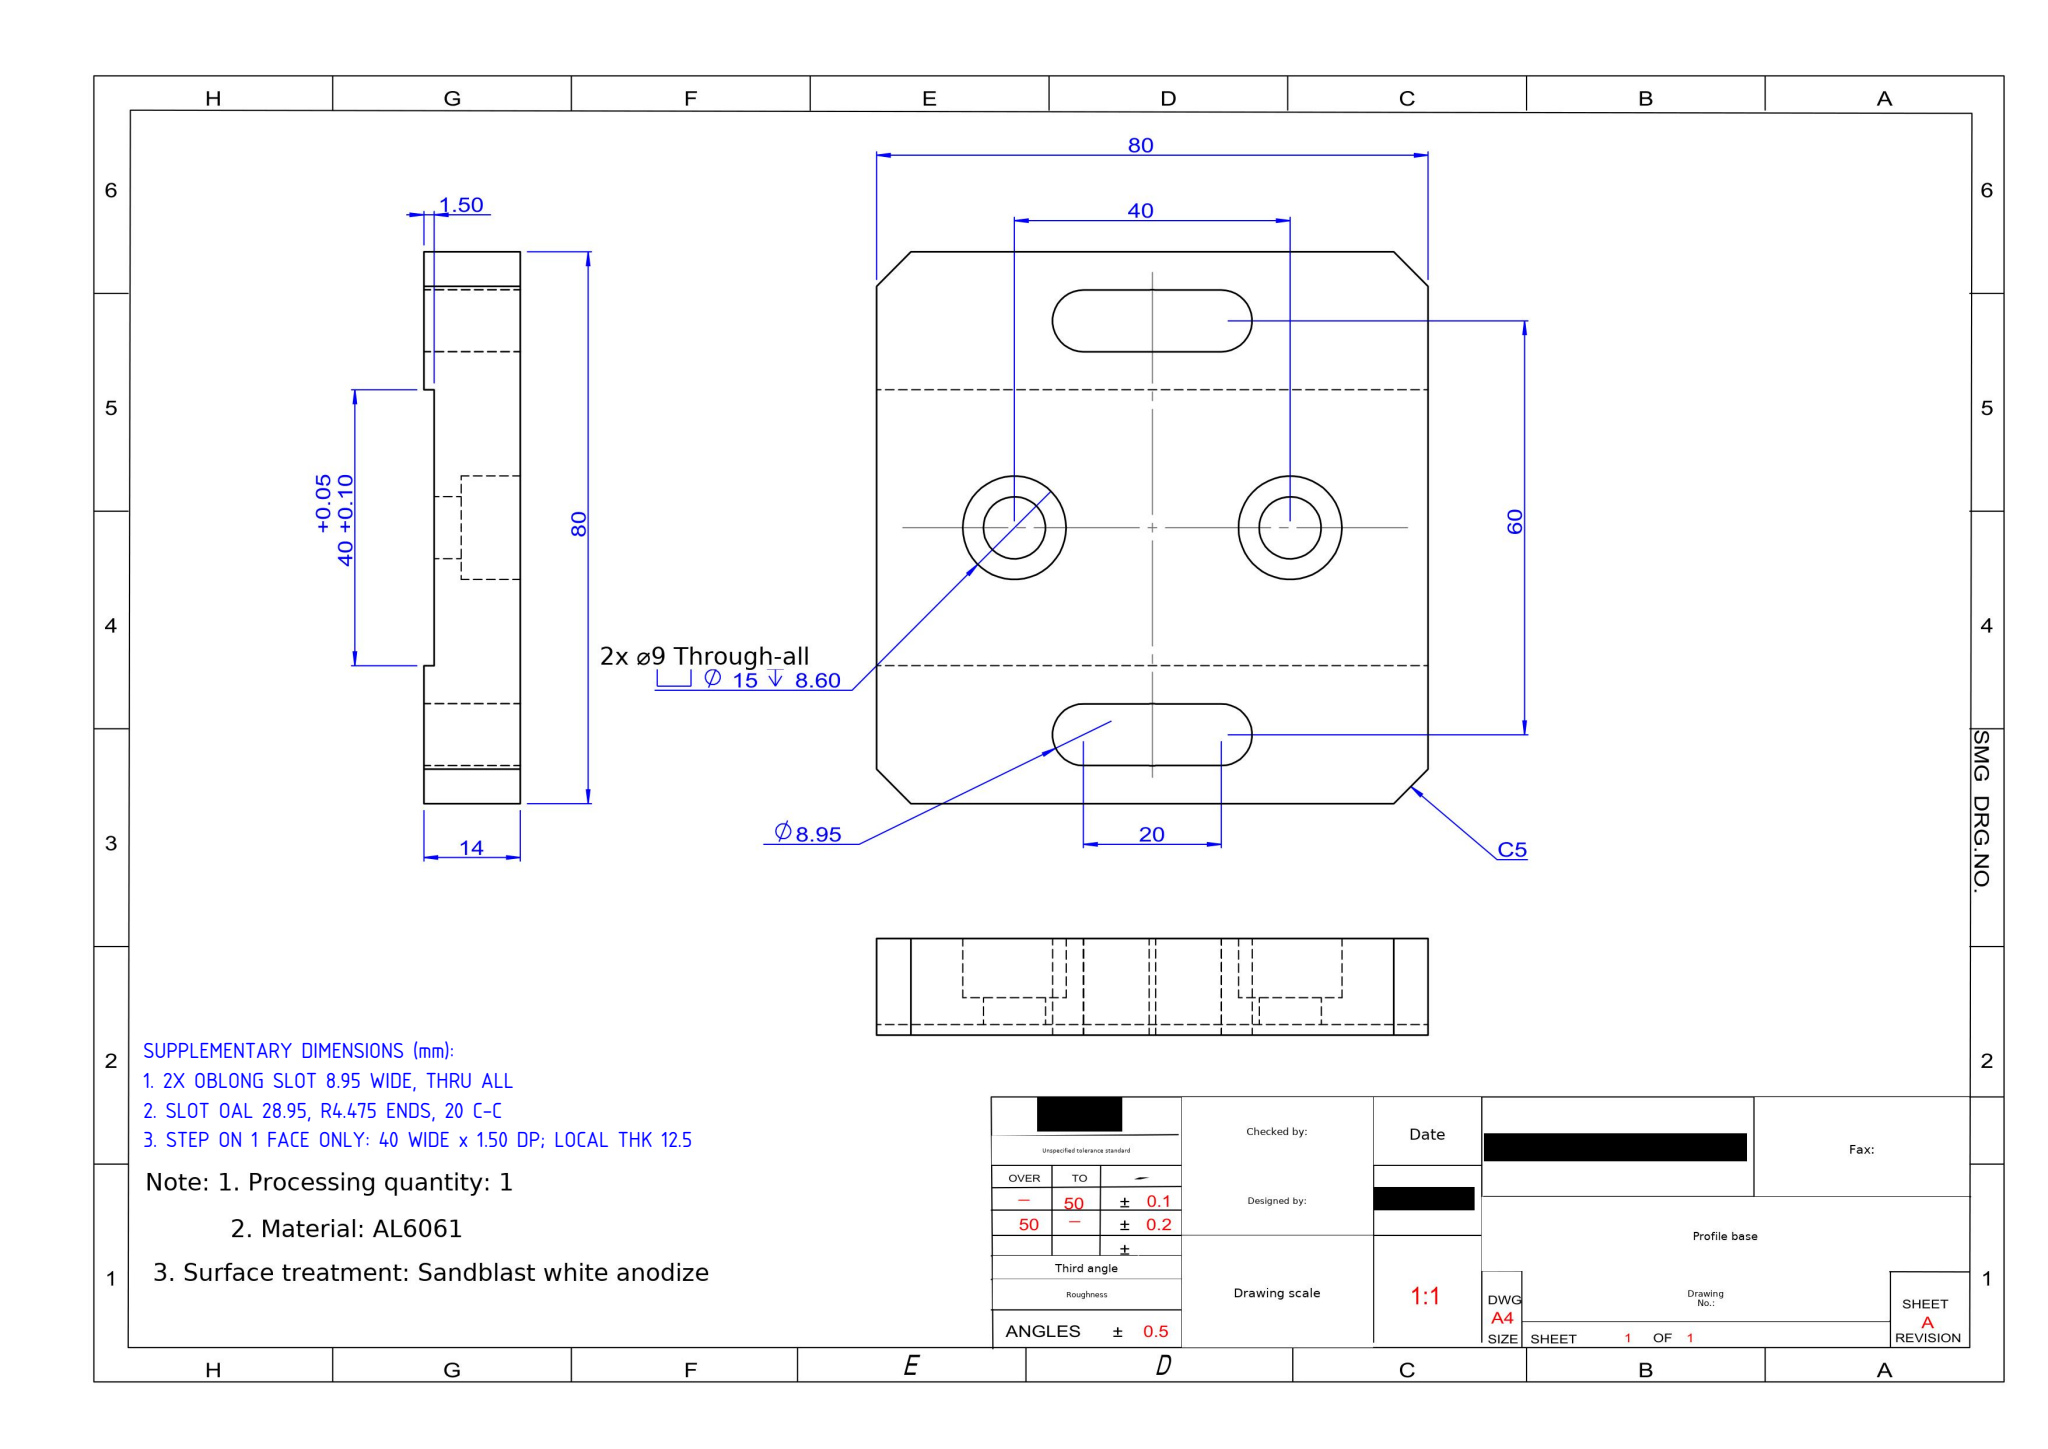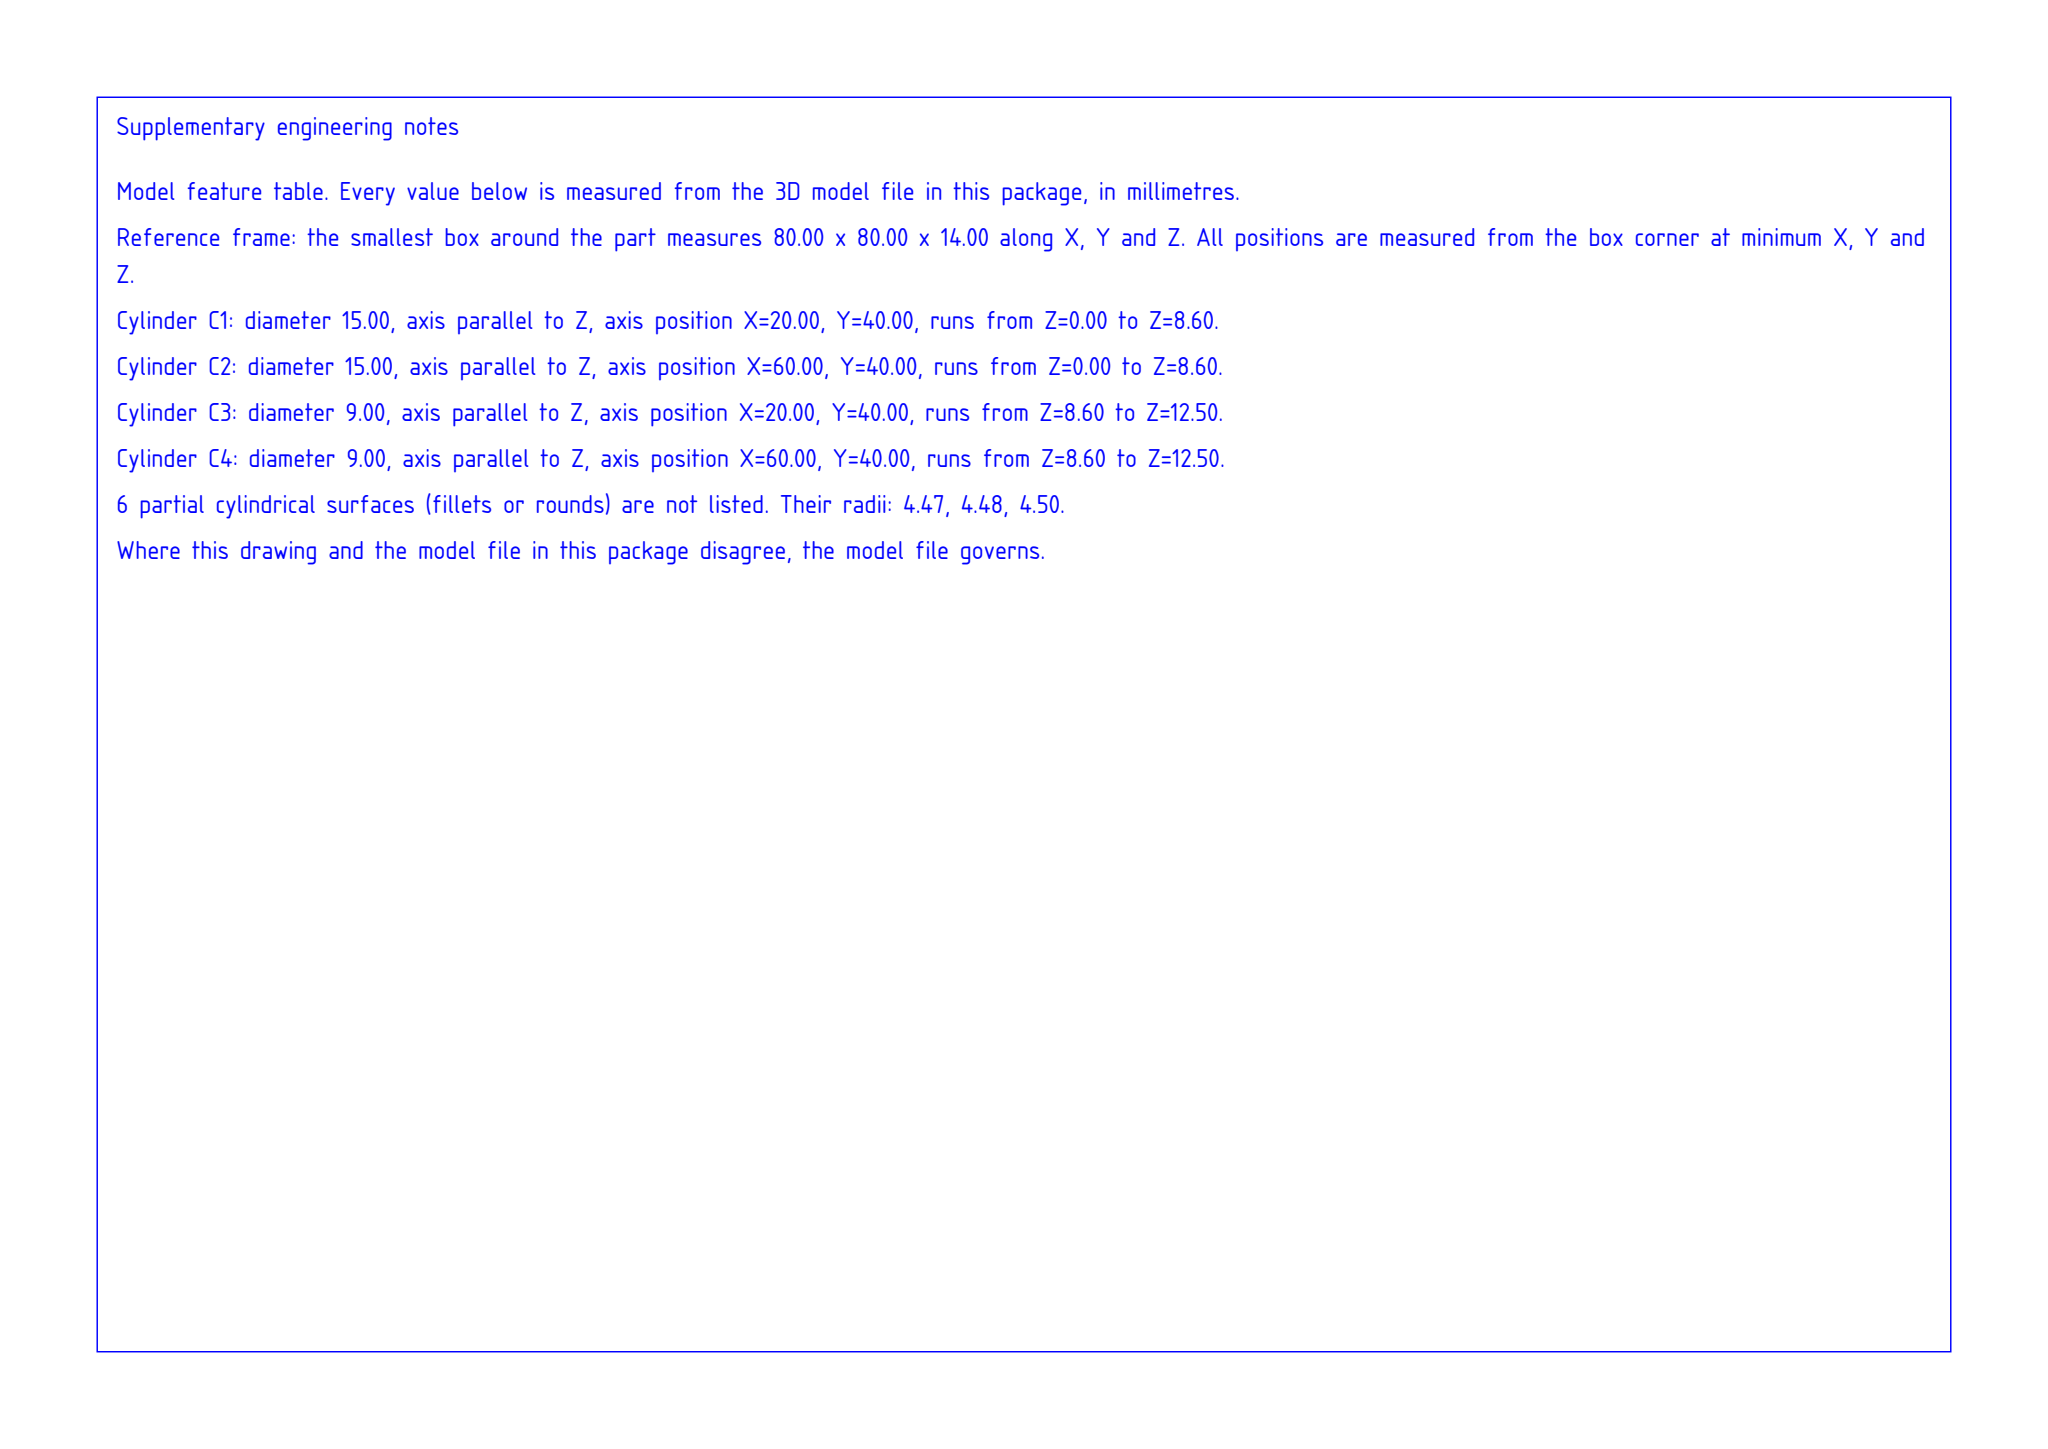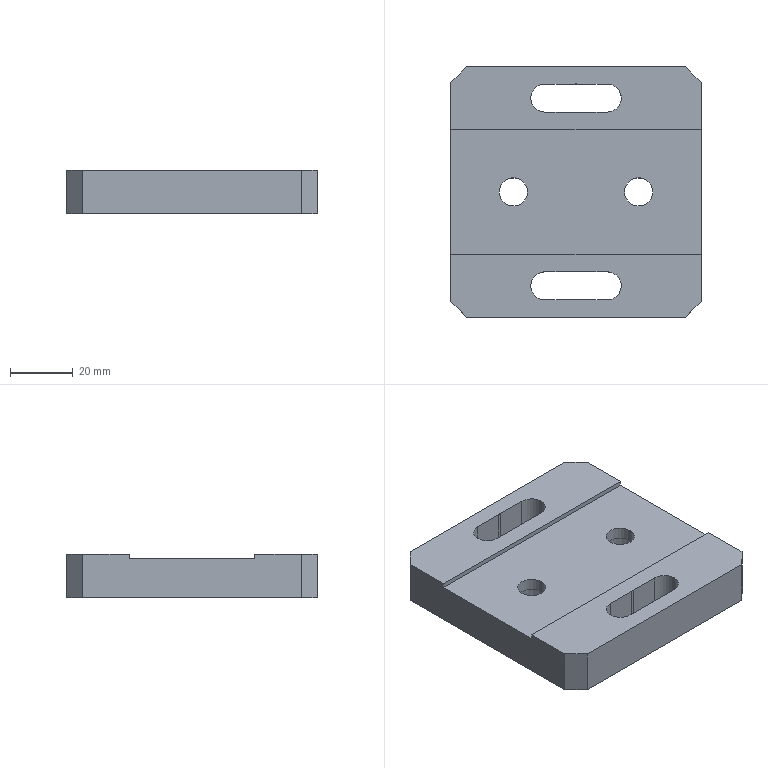Part | SolidWorks | mm | 1 solid | 42 faces | box 80 x 80 x 14 mm | volume 73790 mm3 | plane 24 | cylinder 18 | commonest cylinder face diameters 9 x8 8.95 x6 15 x4